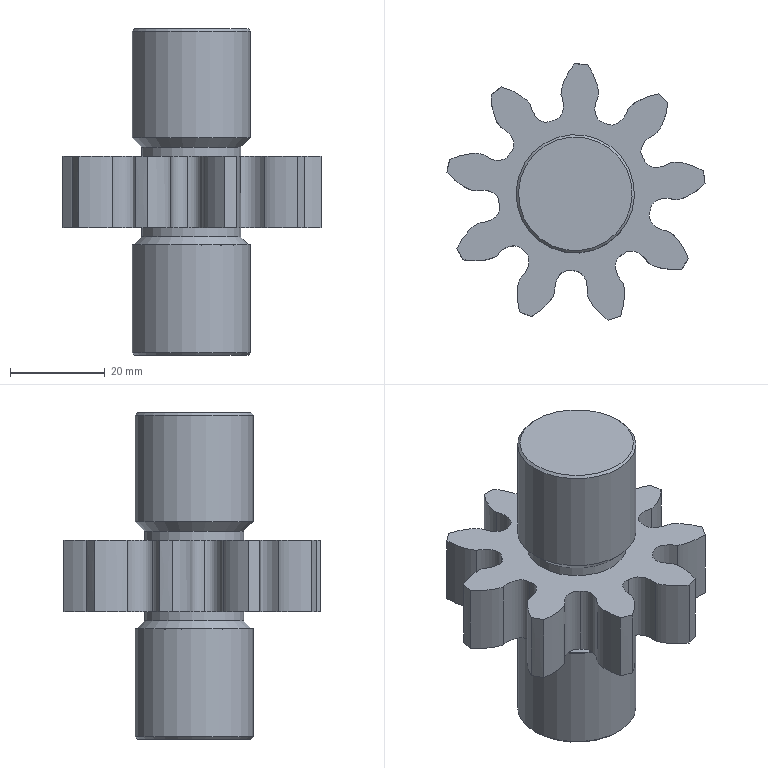Component | NX | CLYB_07_OUTPUTGEARSHAFT | 1 solid | 58 faces | volume 48138 mm3 | spline 36 | other 9 | cone 5 | plane 4 | cylinder 4 | commonest cylinder face diameters 21 x2 25 x2